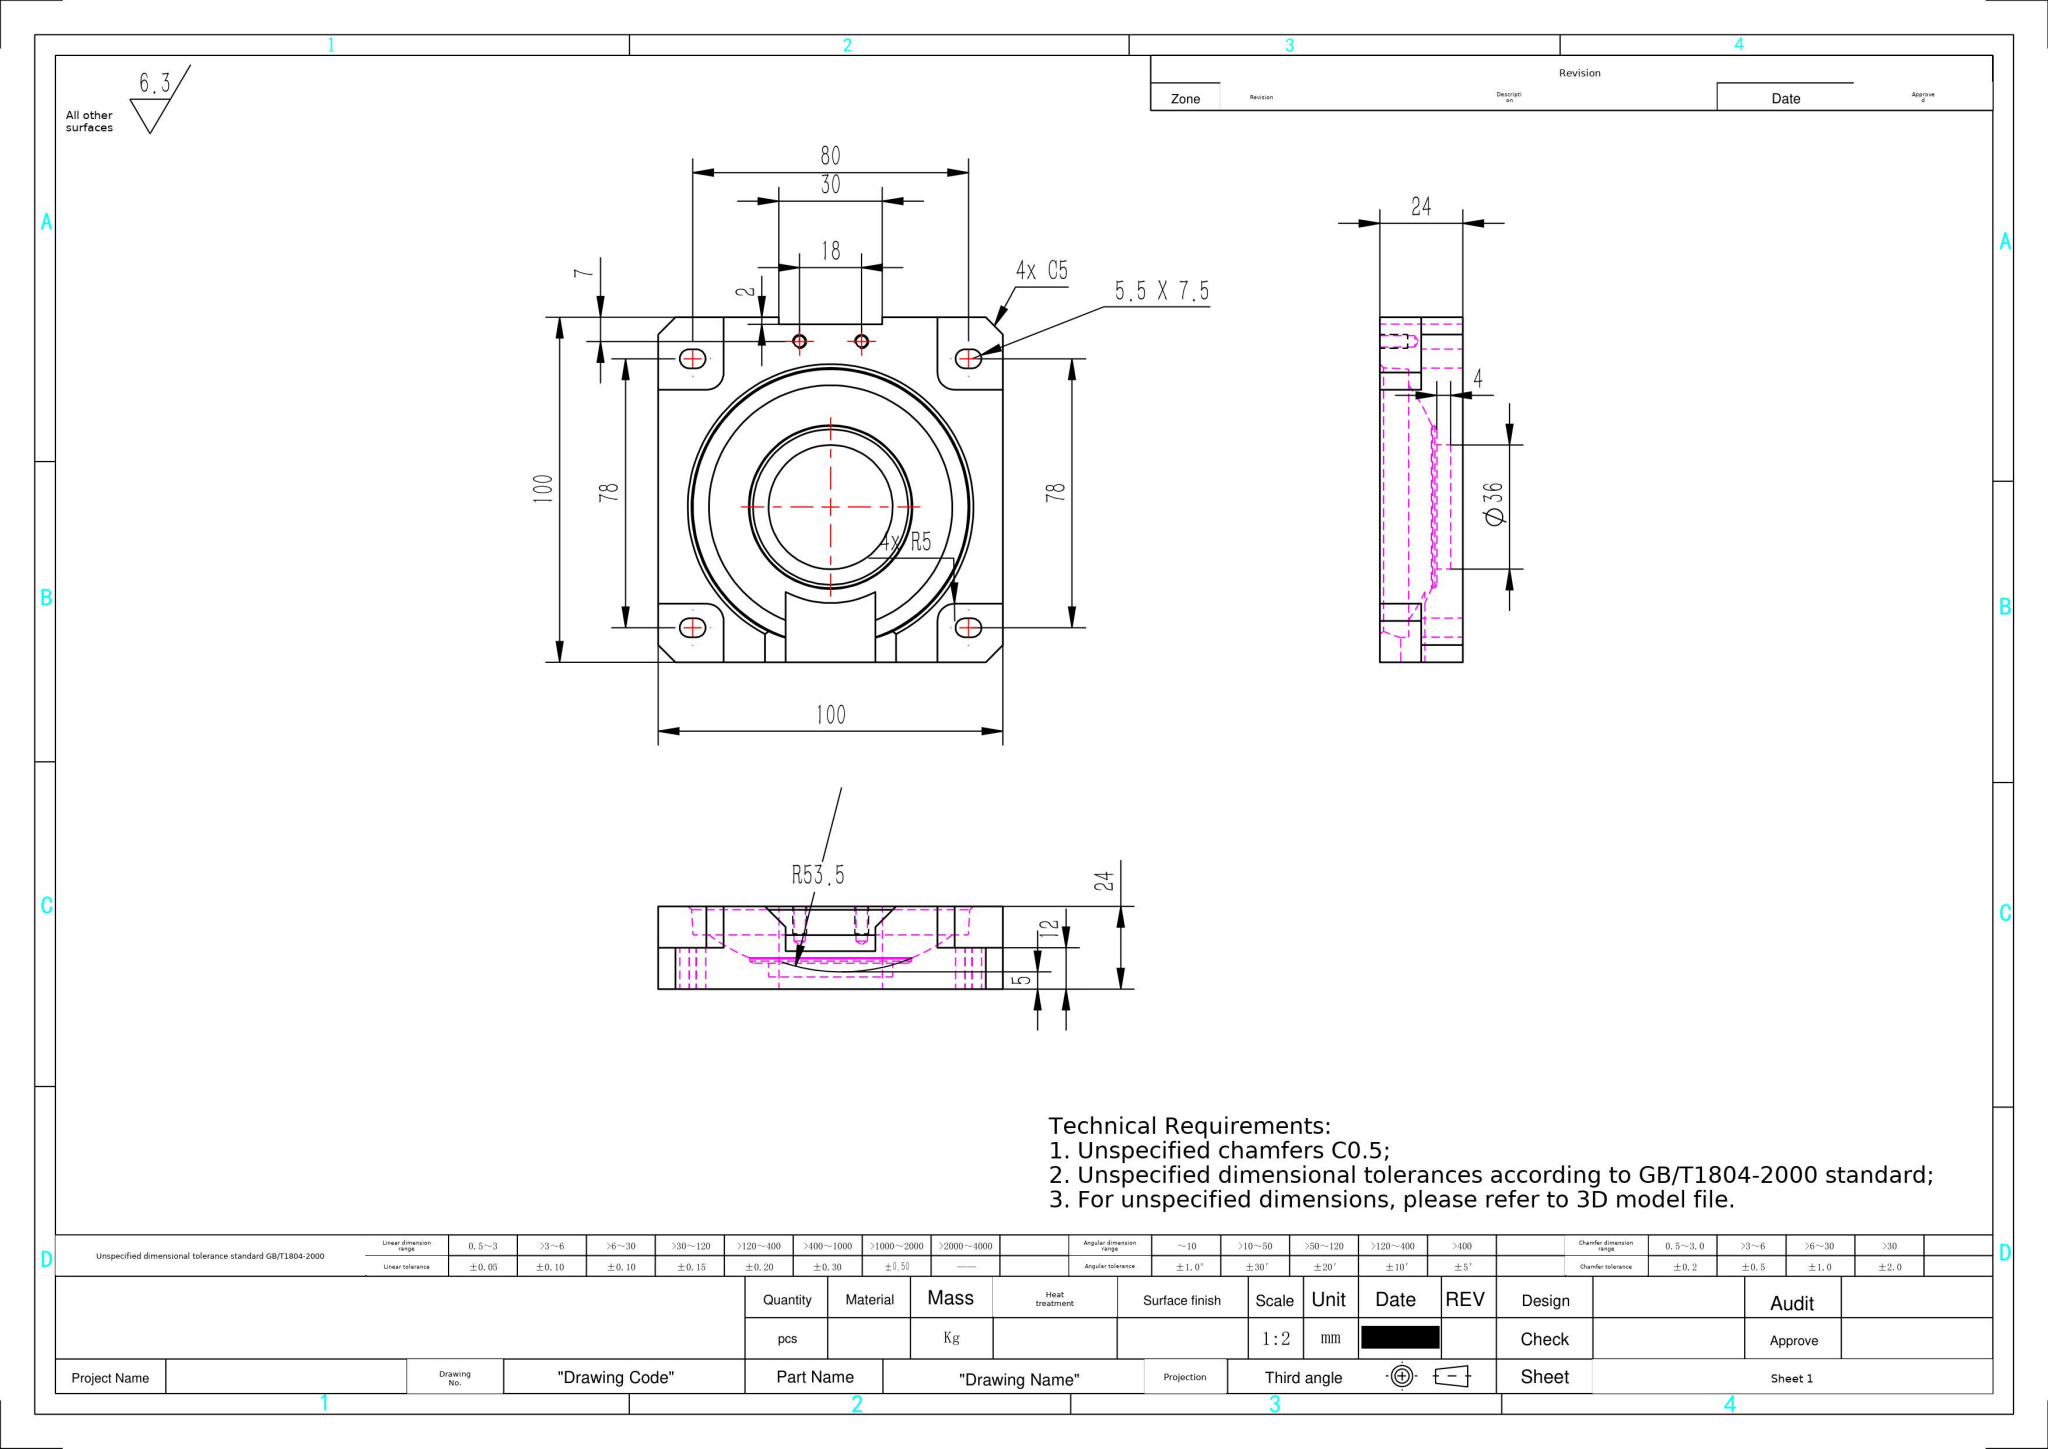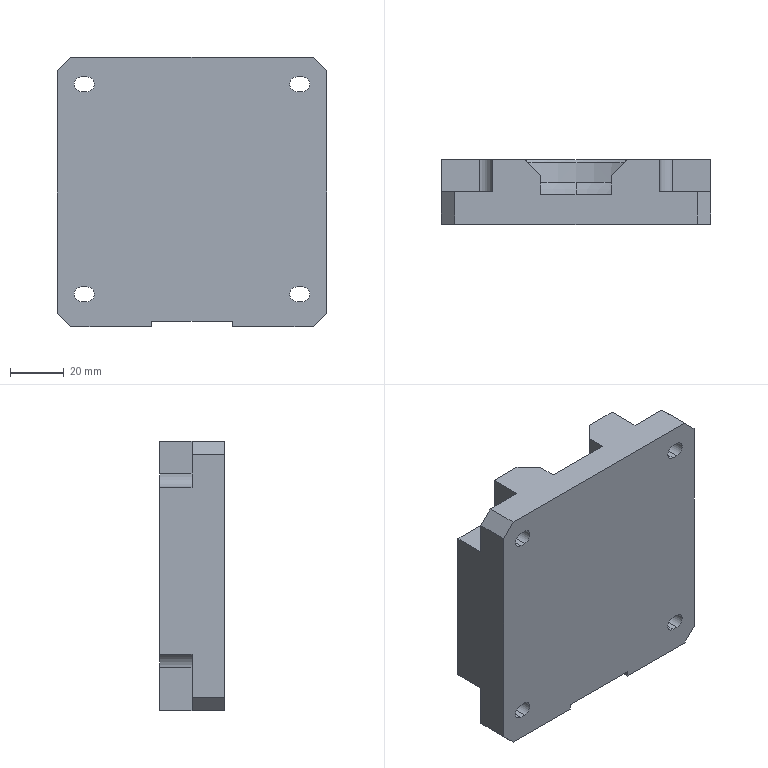Part | SolidWorks | mm | 1 solid | 74 faces | box 100 x 24 x 100 mm | volume 147874 mm3 | plane 42 | cylinder 20 | cone 8 | torus 4 | commonest cylinder face diameters 5.5 x8 3.3 x4 10 x4 47 x2 36 x2